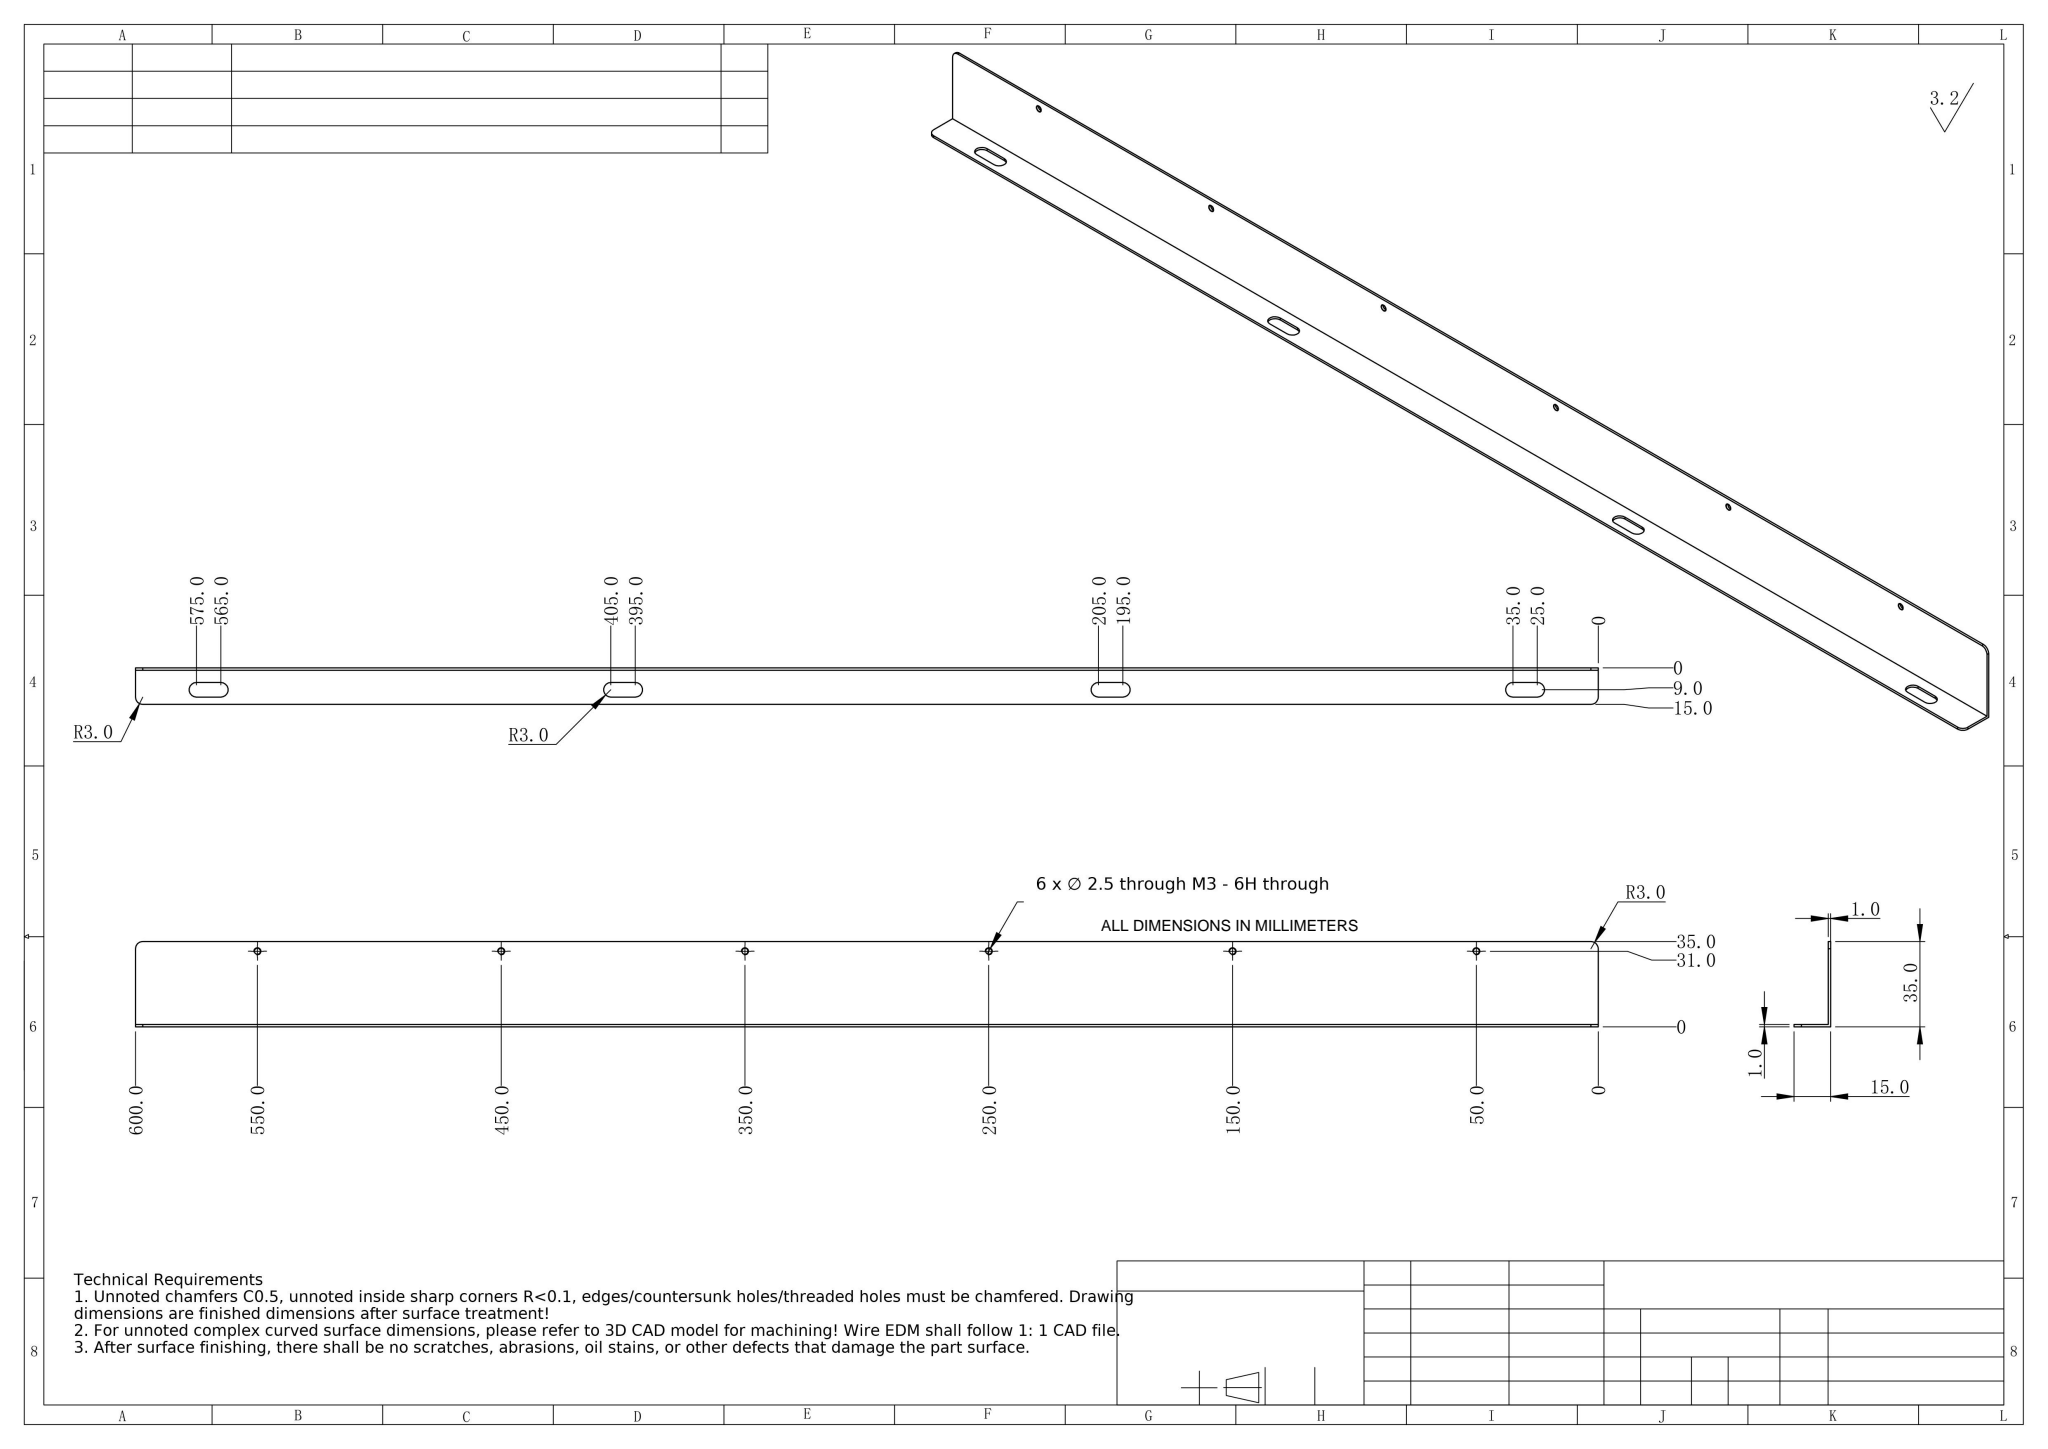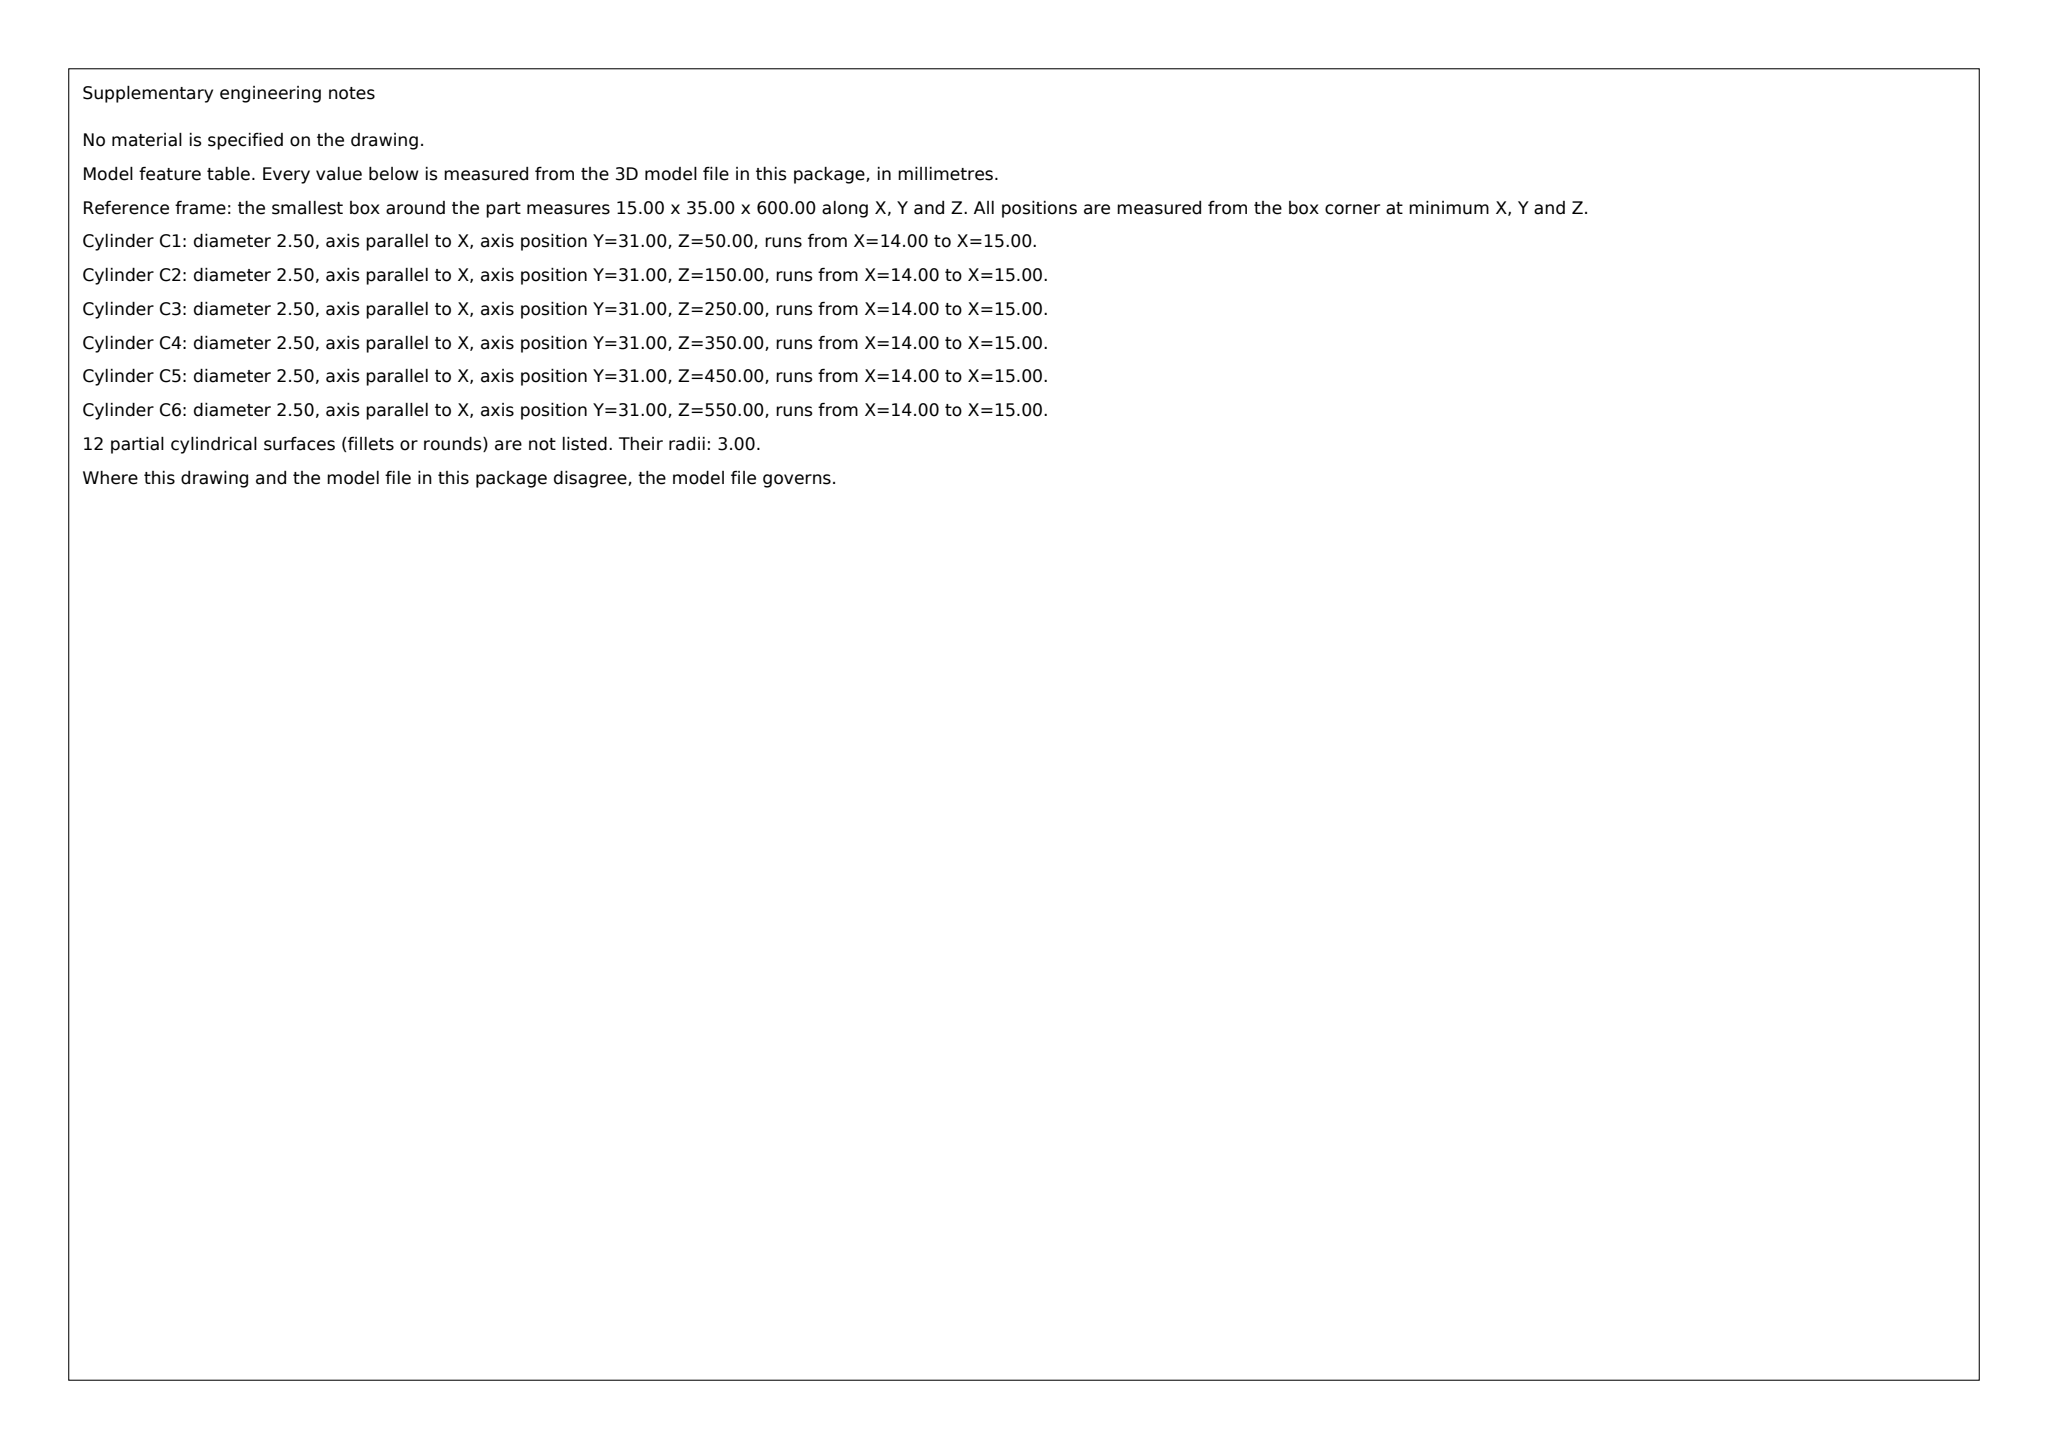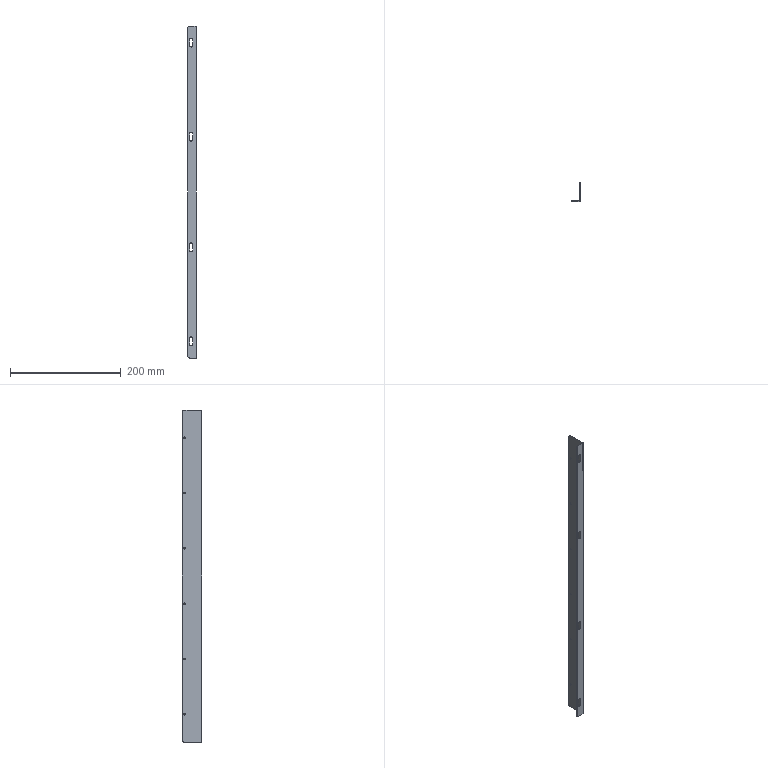Part | SolidWorks | mm | 1 solid | 44 faces | box 15 x 35 x 600 mm | volume 29010 mm3 | cylinder 28 | plane 16 | commonest cylinder face diameters 6 x16 2.5 x12
build123d program:
from build123d import *

# Parameters (mm, degrees)
EXTRUDE_THIN1_DEPTH = 300
FILLET1_R           = 3
M3_TAPPED_HOLE1_D   = 2.5
CUT_EXTRUDE1_DEPTH  = 10


with BuildPart() as part:
    # Sketch1 → Extrude-Thin1 (new, symmetric)
    with BuildSketch(Plane.XY):
        Polygon((0, 0), (0, -35), (-15, -35), (-15, -34), (-1, -34), (-1, 0), align=None)
    extrude(amount=EXTRUDE_THIN1_DEPTH, both=True)

    # Fillet1
    fillet1_edges = [part.edges().sort_by_distance(p)[0] for p in [
        (-0.5, 0, 300),
        (-0.5, 0, -300),
        (-15, -34.5, -300),
        (-15, -34.5, 300),
    ]]
    fillet(fillet1_edges, radius=FILLET1_R)

    # M3 Tapped Hole1 (through all)
    with Locations(Plane.ZY.offset(1)):
        with Locations((-250, -4), (-150, -4), (-50, -4), (50, -4), (150, -4), (250, -4)):
            Hole(M3_TAPPED_HOLE1_D / 2)

    # Sketch4 → Cut-Extrude1 (cut)
    with BuildSketch(Plane.XZ.offset(35)):
        with BuildLine():
            Line((-6, 275), (-6, 265))
            ThreePointArc((-6, 265), (-9, 262), (-12, 265))
            Line((-12, 265), (-12, 275))
            ThreePointArc((-12, 275), (-9, 278), (-6, 275))
        make_face()
        with BuildLine():
            Line((-6, 105), (-6, 95))
            ThreePointArc((-6, 95), (-9, 92), (-12, 95))
            Line((-12, 95), (-12, 105))
            ThreePointArc((-12, 105), (-9, 108), (-6, 105))
        make_face()
        with BuildLine():
            Line((-6, -105), (-6, -95))
            ThreePointArc((-6, -95), (-9, -92), (-12, -95))
            Line((-12, -95), (-12, -105))
            ThreePointArc((-12, -105), (-9, -108), (-6, -105))
        make_face()
        with BuildLine():
            Line((-6, -275), (-6, -265))
            ThreePointArc((-6, -265), (-9, -262), (-12, -265))
            Line((-12, -265), (-12, -275))
            ThreePointArc((-12, -275), (-9, -278), (-6, -275))
        make_face()
    extrude(amount=-CUT_EXTRUDE1_DEPTH, mode=Mode.SUBTRACT)


solid = part.part